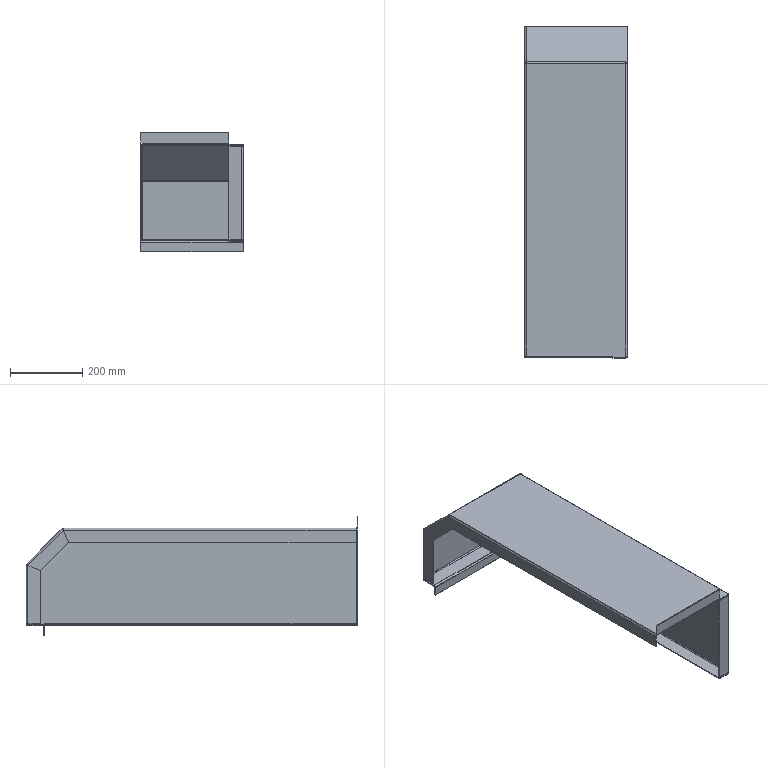Component | NX | SIDE_COLUMN_REAR_LEFT | 1 solid | 93 faces | volume 1337436 mm3 | plane 70 | cylinder 23 | commonest cylinder face diameters 6 x12 10 x11